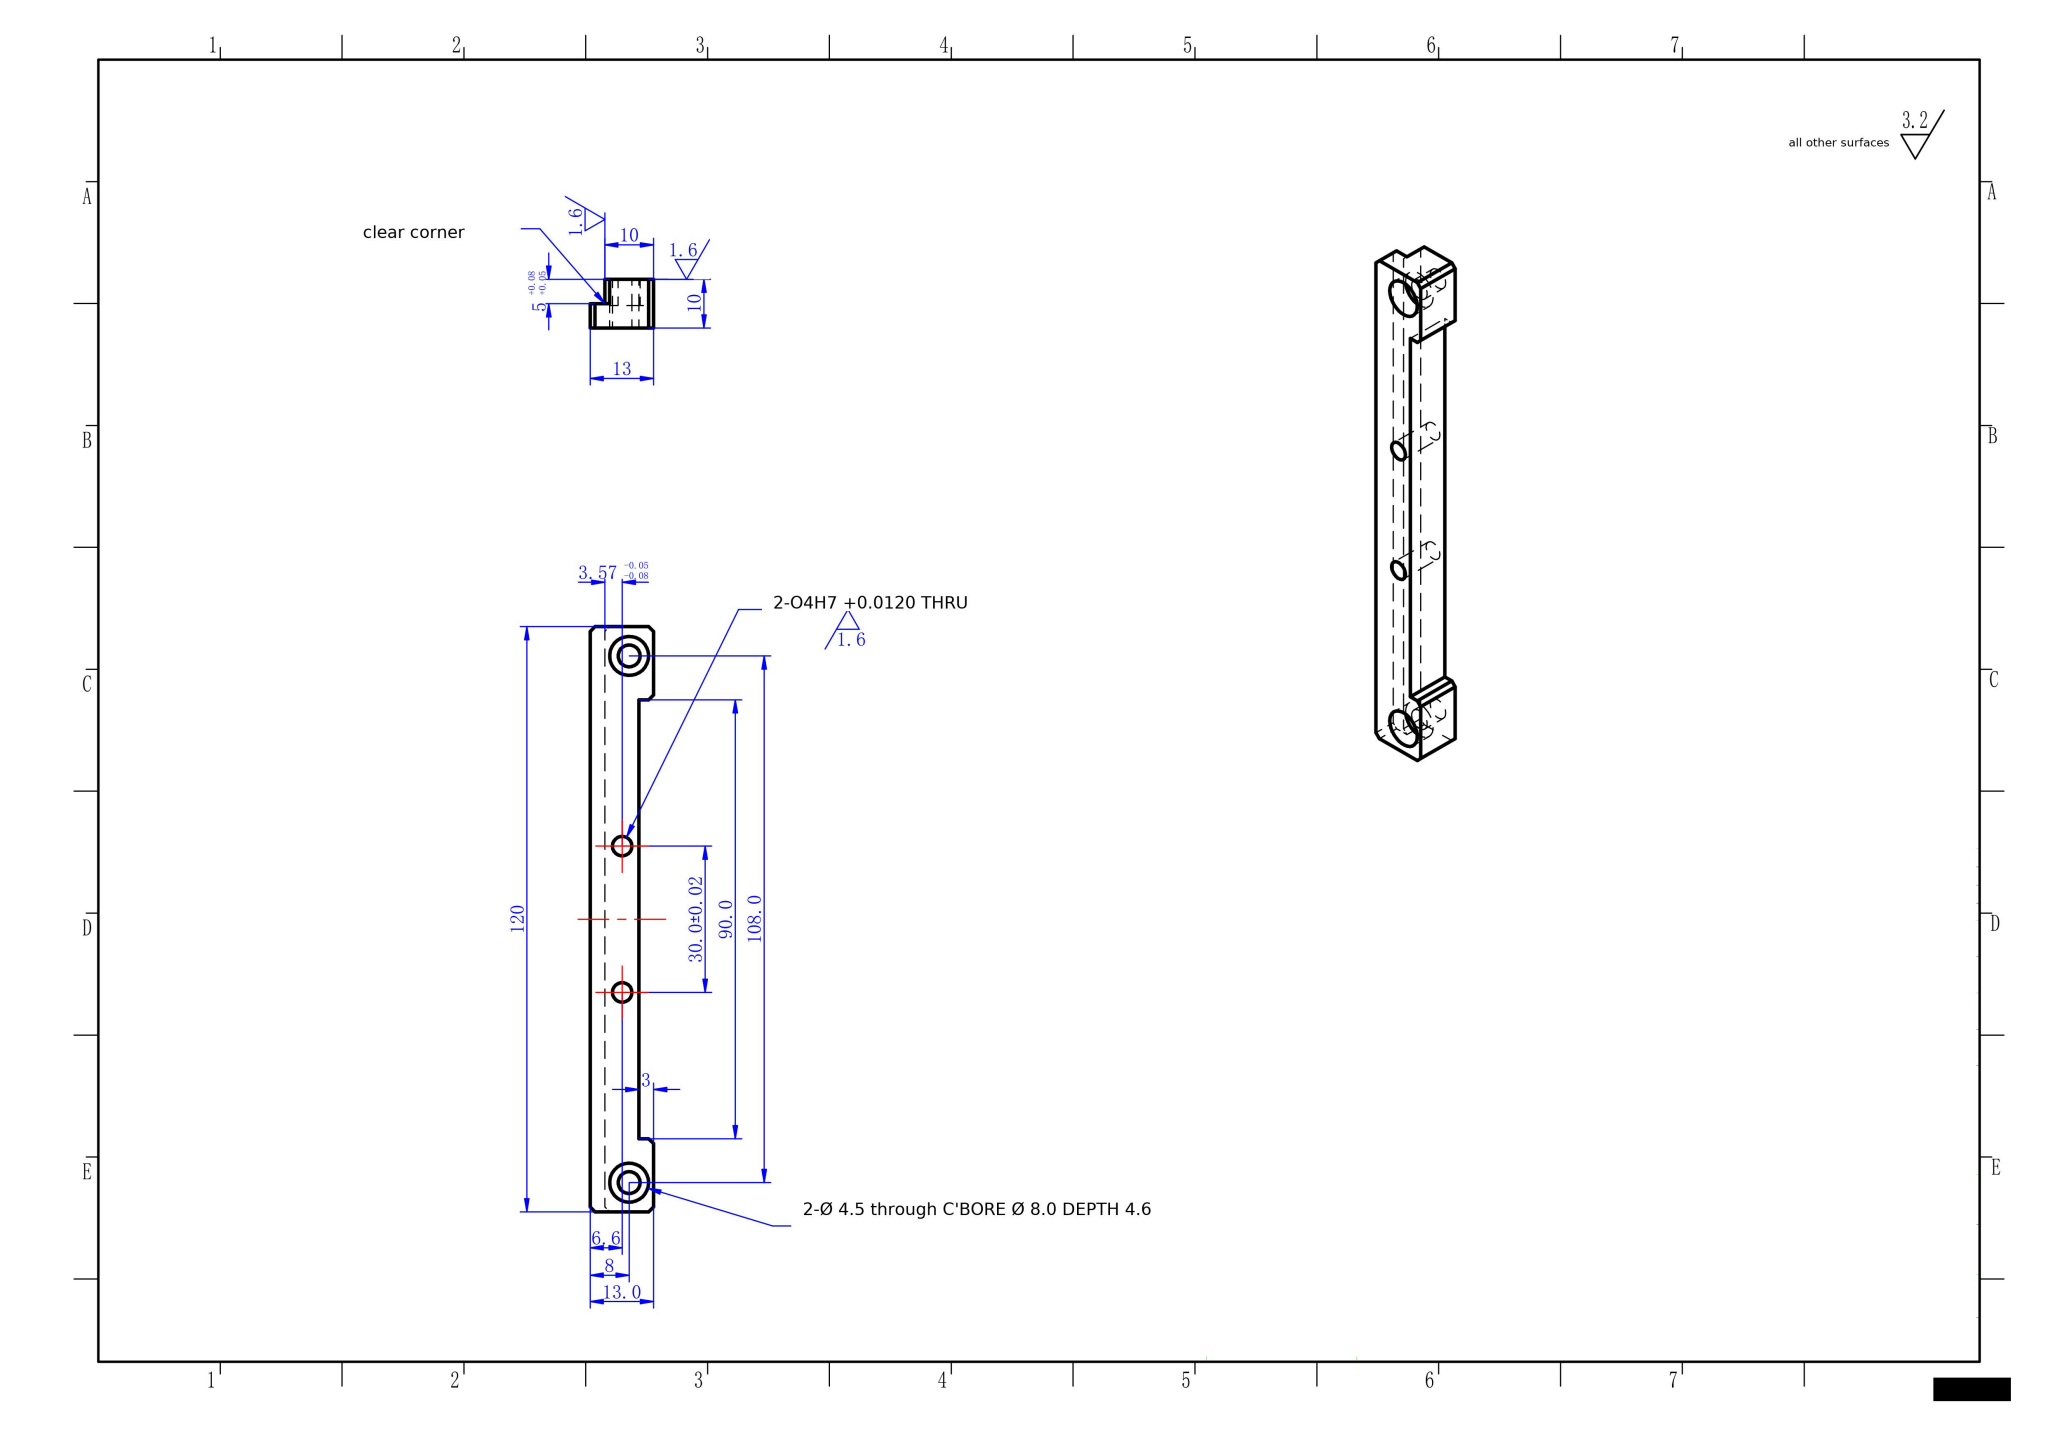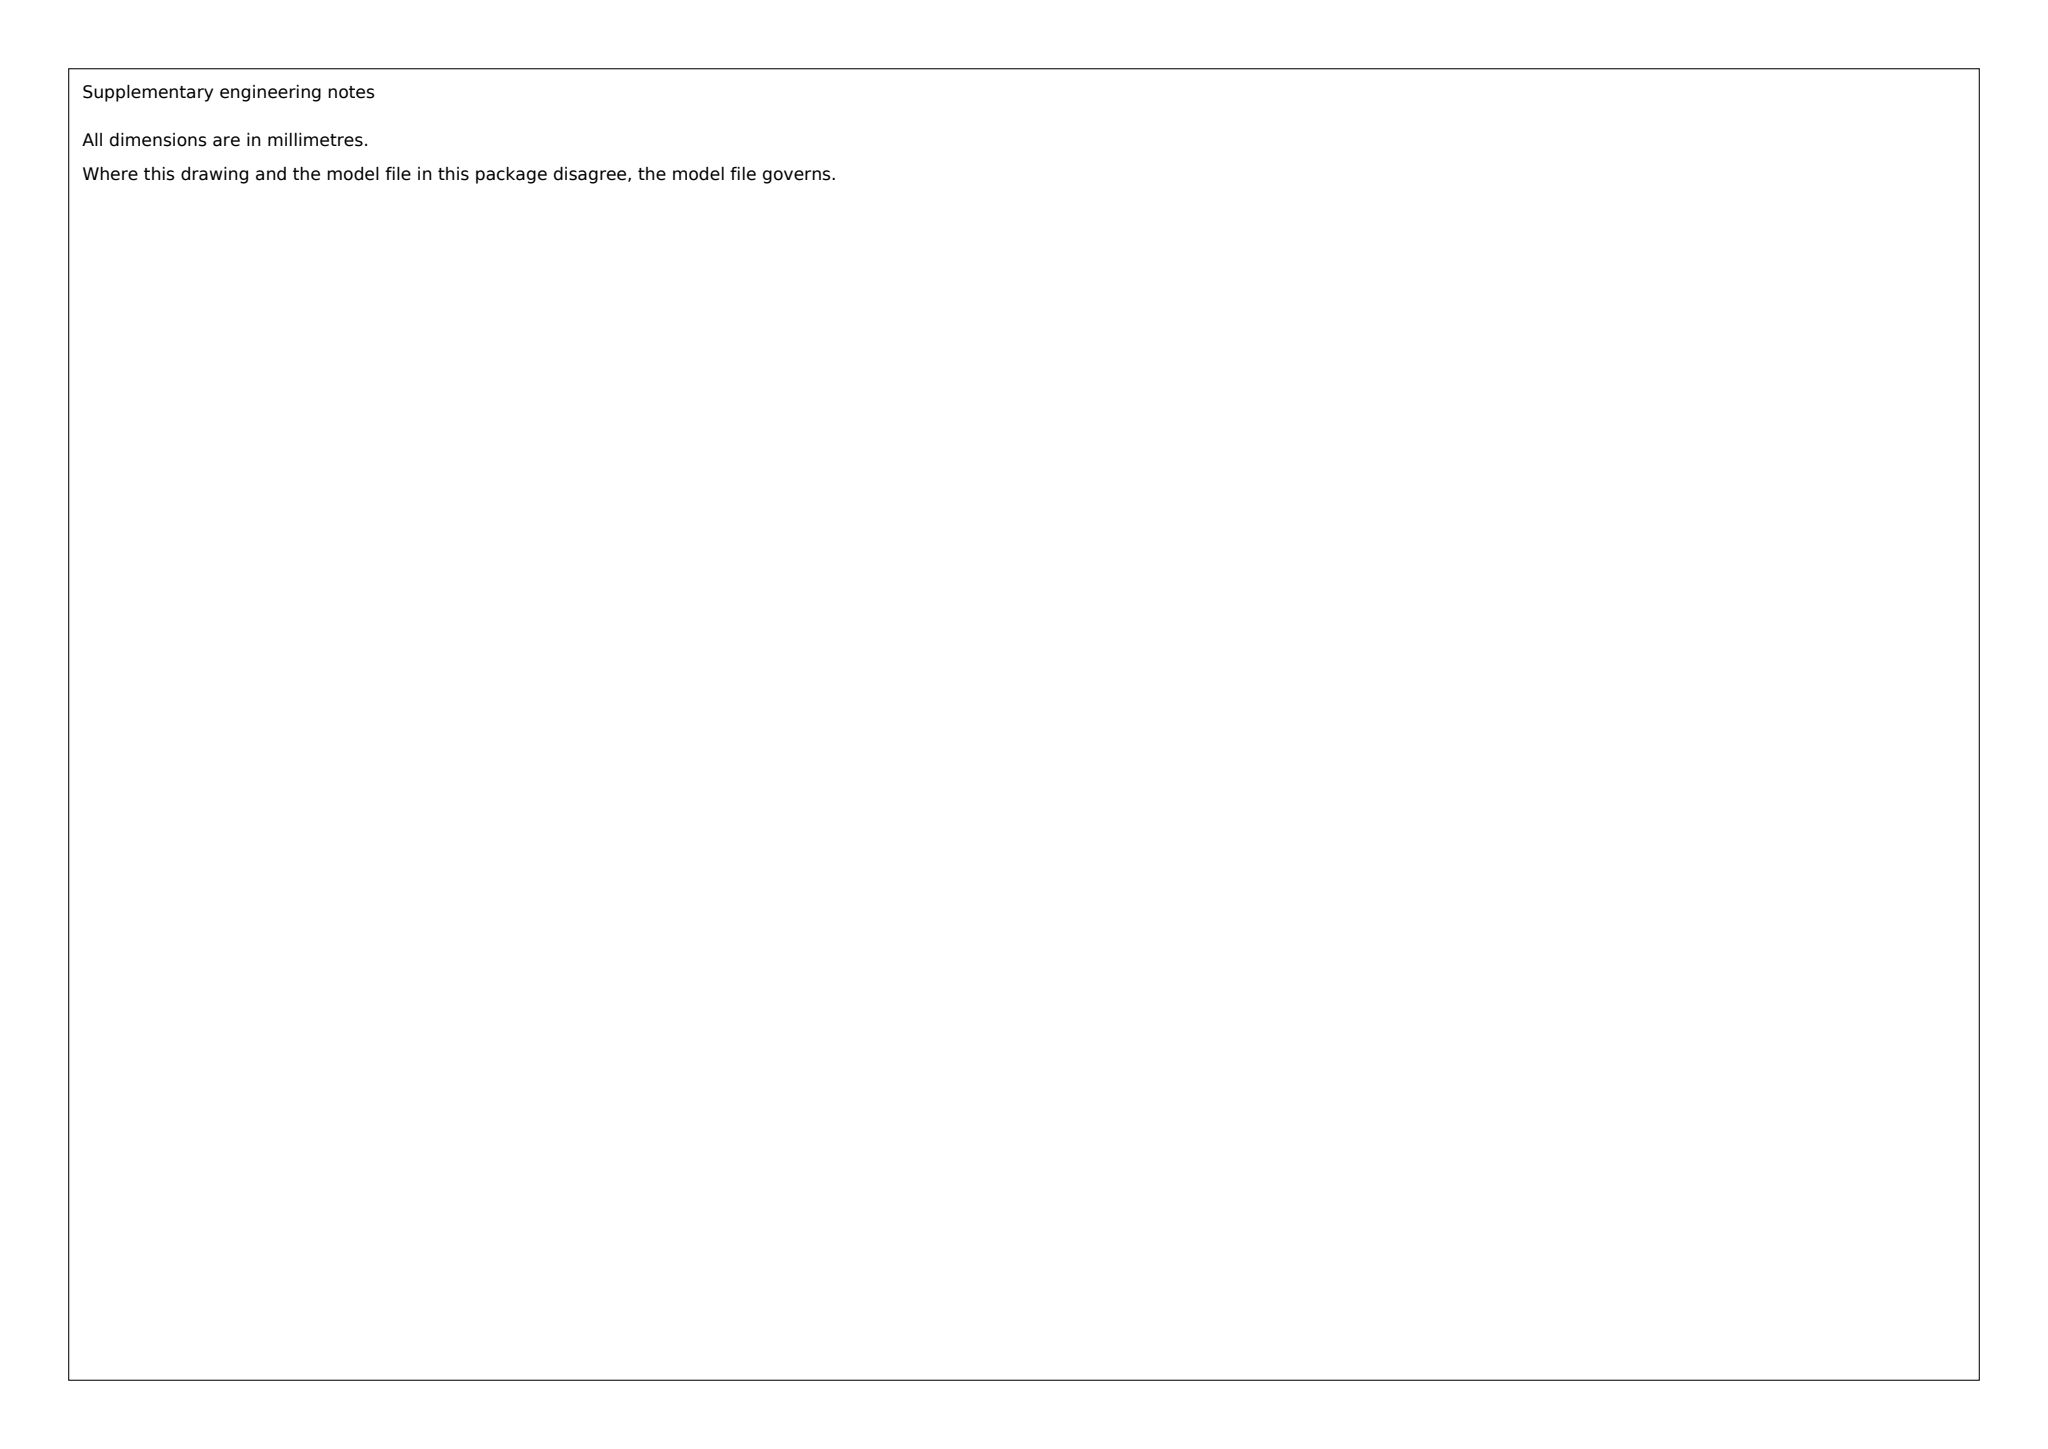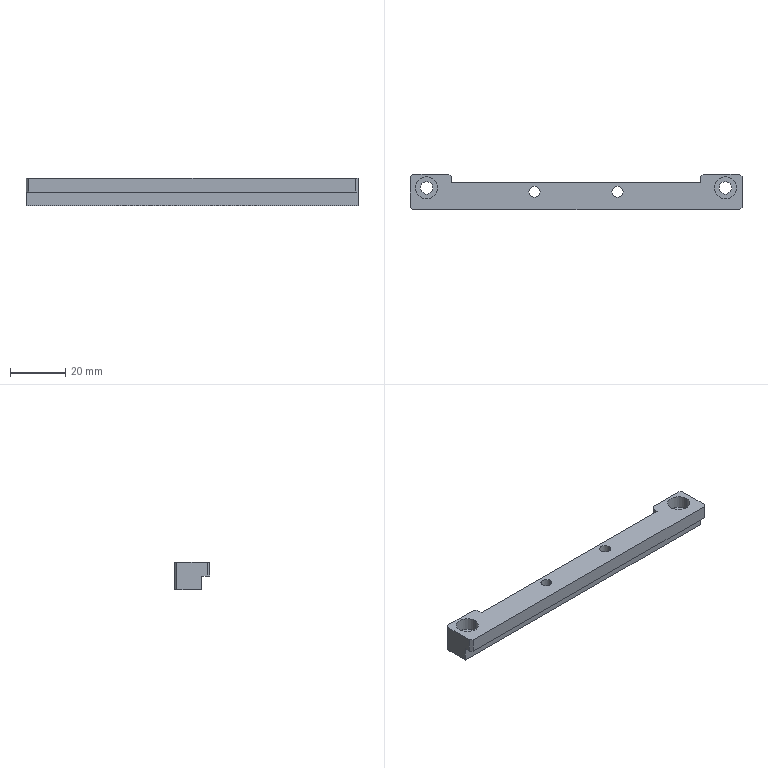Part | SolidWorks | mm | 1 solid | 32 faces | box 120 x 13 x 10 mm | volume 10189 mm3 | plane 20 | cylinder 12 | commonest cylinder face diameters 4 x4 8 x4 4.5 x4